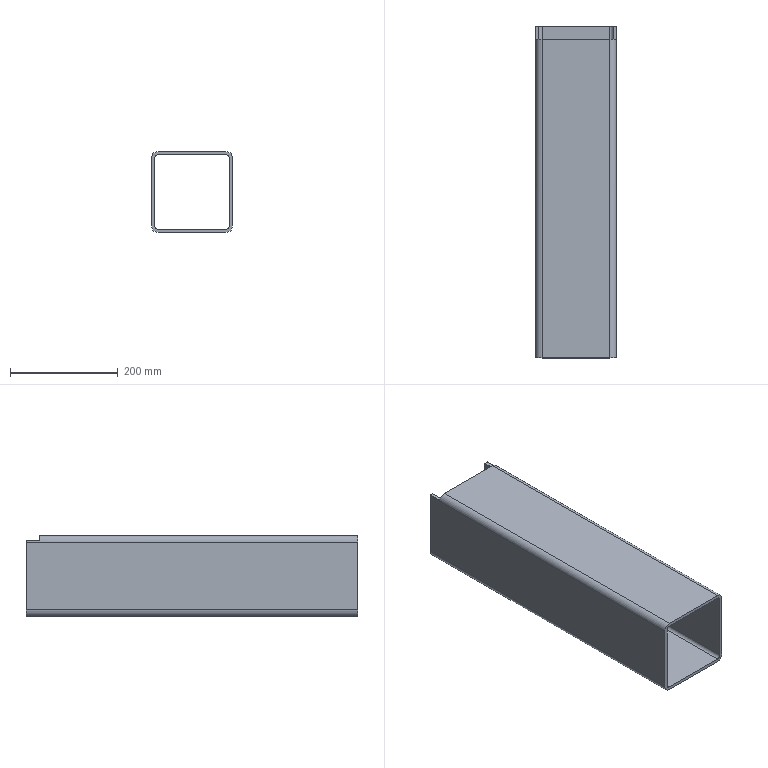Component | SolidWorks | Link2-12 | 1 solid | 21 faces | box 150 x 615 x 150 mm | volume 2045889 mm3 | plane 13 | cylinder 8 | commonest cylinder face diameters 24 x4 12 x4 | material Plain Carbon Steel
build123d program:
from build123d import *

# Parameters (mm, degrees)
BOSS_EXTRUDE1_DEPTH = 615
SKETCH3_W           = 150
SKETCH3_H           = 25
CUT_EXTRUDE1_DEPTH  = 10


with BuildPart() as part:
    # Sketch1 → Boss-Extrude1 (new body)
    with BuildSketch(Plane.XY):
        with BuildLine():
            Line((-63, -75), (63, -75))
            ThreePointArc((63, -75), (71.485, -71.485), (75, -63))
            Line((75, -63), (75, 63))
            ThreePointArc((75, 63), (71.485, 71.485), (63, 75))
            Line((63, 75), (-63, 75))
            ThreePointArc((-63, 75), (-71.485, 71.485), (-75, 63))
            Line((-75, 63), (-75, -63))
            ThreePointArc((-75, -63), (-71.485, -71.485), (-63, -75))
        make_face()
        with BuildLine():
            Line((-63, -69), (63, -69))
            ThreePointArc((63, -69), (67.243, -67.243), (69, -63))
            Line((69, -63), (69, 63))
            ThreePointArc((69, 63), (67.243, 67.243), (63, 69))
            Line((63, 69), (-63, 69))
            ThreePointArc((-63, 69), (-67.243, 67.243), (-69, 63))
            Line((-69, 63), (-69, -63))
            ThreePointArc((-69, -63), (-67.243, -67.243), (-63, -69))
        make_face(mode=Mode.SUBTRACT)
    extrude(amount=BOSS_EXTRUDE1_DEPTH)

    # Sketch3 → Cut-Extrude1 (cut)
    with BuildSketch(Plane(origin=(0, 75, 0), x_dir=(1, 0, 0), z_dir=(0, 1, 0))):
        with Locations((0, -12.5)):
            Rectangle(SKETCH3_W, SKETCH3_H)
    extrude(amount=-CUT_EXTRUDE1_DEPTH, mode=Mode.SUBTRACT)


solid = part.part

# Placed as in the assembly
solid = solid.moved(Location((6192.801, 221.323, 5500.973), (90, 0, 0)))
STEP:
#1=COLOUR_RGB('',0.7922,0.8196,0.9333);
#2=FILL_AREA_STYLE_COLOUR('',#1);
#3=FILL_AREA_STYLE('',(#2));
#4=SURFACE_STYLE_FILL_AREA(#3);
#5=SURFACE_SIDE_STYLE('',(#4));
#6=SURFACE_STYLE_USAGE(.BOTH.,#5);
#7=PRESENTATION_STYLE_ASSIGNMENT((#6));
#8=CARTESIAN_POINT('',(246.757,8.713,219.133));
#9=VERTEX_POINT('',#8);
#10=CARTESIAN_POINT('',(246.514,8.713,219.133));
#11=VERTEX_POINT('',#10);
#12=CARTESIAN_POINT('',(240.858,8.713,219.133));
#13=DIRECTION('',(-1.,0.,0.));
#14=VECTOR('',#13,39.37);
#15=LINE('',#12,#14);
#16=EDGE_CURVE('',#9,#11,#15,.T.);
#17=ORIENTED_EDGE('',*,*,#16,.F.);
#18=CARTESIAN_POINT('',(246.764,8.713,219.054));
#19=VERTEX_POINT('',#18);
#20=CARTESIAN_POINT('',(246.291,8.713,219.054));
#21=DIRECTION('',(0.,-1.,-0.));
#22=DIRECTION('',(1.,0.,0.));
#23=AXIS2_PLACEMENT_3D('',#20,#21,#22);
#24=CIRCLE('',#23,0.4724);
#25=EDGE_CURVE('',#19,#9,#24,.T.);
#26=ORIENTED_EDGE('',*,*,#25,.F.);
#27=CARTESIAN_POINT('',(246.764,8.713,214.093));
#28=VERTEX_POINT('',#27);
#29=CARTESIAN_POINT('',(246.764,8.713,219.054));
#30=DIRECTION('',(0.,0.,-1.));
#31=VECTOR('',#30,39.37);
#32=LINE('',#29,#31);
#33=EDGE_CURVE('',#19,#28,#32,.T.);
#34=ORIENTED_EDGE('',*,*,#33,.T.);
#35=CARTESIAN_POINT('',(246.291,8.713,213.621));
#36=VERTEX_POINT('',#35);
#37=CARTESIAN_POINT('',(246.291,8.713,214.093));
#38=DIRECTION('',(0.,-1.,-0.));
#39=DIRECTION('',(1.,0.,0.));
#40=AXIS2_PLACEMENT_3D('',#37,#38,#39);
#41=CIRCLE('',#40,0.4724);
#42=EDGE_CURVE('',#36,#28,#41,.T.);
#43=ORIENTED_EDGE('',*,*,#42,.F.);
#44=CARTESIAN_POINT('',(241.331,8.713,213.621));
#45=VERTEX_POINT('',#44);
#46=CARTESIAN_POINT('',(241.331,8.713,213.621));
#47=DIRECTION('',(1.,0.,0.));
#48=VECTOR('',#47,39.37);
#49=LINE('',#46,#48);
#50=EDGE_CURVE('',#45,#36,#49,.T.);
#51=ORIENTED_EDGE('',*,*,#50,.F.);
#52=CARTESIAN_POINT('',(240.858,8.713,214.093));
#53=VERTEX_POINT('',#52);
#54=CARTESIAN_POINT('',(241.331,8.713,214.093));
#55=DIRECTION('',(0.,-1.,-0.));
#56=DIRECTION('',(1.,0.,0.));
#57=AXIS2_PLACEMENT_3D('',#54,#55,#56);
#58=CIRCLE('',#57,0.4724);
#59=EDGE_CURVE('',#53,#45,#58,.T.);
#60=ORIENTED_EDGE('',*,*,#59,.F.);
#61=CARTESIAN_POINT('',(240.858,8.713,219.054));
#62=VERTEX_POINT('',#61);
#63=CARTESIAN_POINT('',(240.858,8.713,214.093));
#64=DIRECTION('',(0.,-0.,1.));
#65=VECTOR('',#64,39.37);
#66=LINE('',#63,#65);
#67=EDGE_CURVE('',#53,#62,#66,.T.);
#68=ORIENTED_EDGE('',*,*,#67,.T.);
#69=CARTESIAN_POINT('',(240.865,8.713,219.133));
#70=VERTEX_POINT('',#69);
#71=CARTESIAN_POINT('',(241.331,8.713,219.054));
#72=DIRECTION('',(0.,-1.,-0.));
#73=DIRECTION('',(1.,0.,0.));
#74=AXIS2_PLACEMENT_3D('',#71,#72,#73);
#75=CIRCLE('',#74,0.4724);
#76=EDGE_CURVE('',#70,#62,#75,.T.);
#77=ORIENTED_EDGE('',*,*,#76,.F.);
#78=CARTESIAN_POINT('',(241.108,8.713,219.133));
#79=VERTEX_POINT('',#78);
#80=CARTESIAN_POINT('',(240.858,8.713,219.133));
#81=DIRECTION('',(-1.,0.,0.));
#82=VECTOR('',#81,39.37);
#83=LINE('',#80,#82);
#84=EDGE_CURVE('',#79,#70,#83,.T.);
#85=ORIENTED_EDGE('',*,*,#84,.F.);
#86=CARTESIAN_POINT('',(241.095,8.713,219.054));
#87=VERTEX_POINT('',#86);
#88=CARTESIAN_POINT('',(241.331,8.713,219.054));
#89=DIRECTION('',(0.,-1.,-0.));
#90=DIRECTION('',(1.,0.,0.));
#91=AXIS2_PLACEMENT_3D('',#88,#89,#90);
#92=CIRCLE('',#91,0.2362);
#93=EDGE_CURVE('',#79,#87,#92,.T.);
#94=ORIENTED_EDGE('',*,*,#93,.T.);
#95=CARTESIAN_POINT('',(241.095,8.713,214.093));
#96=VERTEX_POINT('',#95);
#97=CARTESIAN_POINT('',(241.095,8.713,214.093));
#98=DIRECTION('',(0.,-0.,1.));
#99=VECTOR('',#98,39.37);
#100=LINE('',#97,#99);
#101=EDGE_CURVE('',#96,#87,#100,.T.);
#102=ORIENTED_EDGE('',*,*,#101,.F.);
#103=CARTESIAN_POINT('',(241.331,8.713,213.857));
#104=VERTEX_POINT('',#103);
#105=CARTESIAN_POINT('',(241.331,8.713,214.093));
#106=DIRECTION('',(0.,-1.,-0.));
#107=DIRECTION('',(1.,0.,0.));
#108=AXIS2_PLACEMENT_3D('',#105,#106,#107);
#109=CIRCLE('',#108,0.2362);
#110=EDGE_CURVE('',#96,#104,#109,.T.);
#111=ORIENTED_EDGE('',*,*,#110,.T.);
#112=CARTESIAN_POINT('',(246.291,8.713,213.857));
#113=VERTEX_POINT('',#112);
#114=CARTESIAN_POINT('',(241.331,8.713,213.857));
#115=DIRECTION('',(1.,0.,0.));
#116=VECTOR('',#115,39.37);
#117=LINE('',#114,#116);
#118=EDGE_CURVE('',#104,#113,#117,.T.);
#119=ORIENTED_EDGE('',*,*,#118,.T.);
#120=CARTESIAN_POINT('',(246.528,8.713,214.093));
#121=VERTEX_POINT('',#120);
#122=CARTESIAN_POINT('',(246.291,8.713,214.093));
#123=DIRECTION('',(0.,-1.,-0.));
#124=DIRECTION('',(1.,0.,0.));
#125=AXIS2_PLACEMENT_3D('',#122,#123,#124);
#126=CIRCLE('',#125,0.2362);
#127=EDGE_CURVE('',#113,#121,#126,.T.);
#128=ORIENTED_EDGE('',*,*,#127,.T.);
#129=CARTESIAN_POINT('',(246.528,8.713,219.054));
#130=VERTEX_POINT('',#129);
#131=CARTESIAN_POINT('',(246.528,8.713,219.054));
#132=DIRECTION('',(0.,0.,-1.));
#133=VECTOR('',#132,39.37);
#134=LINE('',#131,#133);
#135=EDGE_CURVE('',#130,#121,#134,.T.);
#136=ORIENTED_EDGE('',*,*,#135,.F.);
#137=CARTESIAN_POINT('',(246.291,8.713,219.054));
#138=DIRECTION('',(0.,-1.,-0.));
#139=DIRECTION('',(1.,0.,0.));
#140=AXIS2_PLACEMENT_3D('',#137,#138,#139);
#141=CIRCLE('',#140,0.2362);
#142=EDGE_CURVE('',#130,#11,#141,.T.);
#143=ORIENTED_EDGE('',*,*,#142,.T.);
#144=EDGE_LOOP('',(#17,#26,#34,#43,#51,#60,#68,#77,#85,#94,#102,#111,#119,#128,#136,#143));
#145=FACE_OUTER_BOUND('',#144,.T.);
#146=CARTESIAN_POINT('',(246.291,8.713,219.054));
#147=DIRECTION('',(0.,-1.,-0.));
#148=DIRECTION('',(1.,0.,0.));
#149=AXIS2_PLACEMENT_3D('',#146,#147,#148);
#150=PLANE('',#149);
#151=ADVANCED_FACE('',(#145),#150,.F.);
#152=CARTESIAN_POINT('',(246.764,-15.499,219.054));
#153=VERTEX_POINT('',#152);
#154=CARTESIAN_POINT('',(246.291,-15.499,219.527));
#155=VERTEX_POINT('',#154);
#156=CARTESIAN_POINT('',(246.291,-15.499,219.054));
#157=DIRECTION('',(0.,-1.,-0.));
#158=DIRECTION('',(1.,0.,0.));
#159=AXIS2_PLACEMENT_3D('',#156,#157,#158);
#160=CIRCLE('',#159,0.4724);
#161=EDGE_CURVE('',#153,#155,#160,.T.);
#162=ORIENTED_EDGE('',*,*,#161,.T.);
#163=CARTESIAN_POINT('',(241.331,-15.499,219.527));
#164=VERTEX_POINT('',#163);
#165=CARTESIAN_POINT('',(246.291,-15.499,219.527));
#166=DIRECTION('',(-1.,0.,0.));
#167=VECTOR('',#166,39.37);
#168=LINE('',#165,#167);
#169=EDGE_CURVE('',#155,#164,#168,.T.);
#170=ORIENTED_EDGE('',*,*,#169,.T.);
#171=CARTESIAN_POINT('',(240.858,-15.499,219.054));
#172=VERTEX_POINT('',#171);
#173=CARTESIAN_POINT('',(241.331,-15.499,219.054));
#174=DIRECTION('',(0.,-1.,-0.));
#175=DIRECTION('',(1.,0.,0.));
#176=AXIS2_PLACEMENT_3D('',#173,#174,#175);
#177=CIRCLE('',#176,0.4724);
#178=EDGE_CURVE('',#164,#172,#177,.T.);
#179=ORIENTED_EDGE('',*,*,#178,.T.);
#180=CARTESIAN_POINT('',(240.858,-15.499,214.093));
#181=VERTEX_POINT('',#180);
#182=CARTESIAN_POINT('',(240.858,-15.499,214.093));
#183=DIRECTION('',(0.,-0.,1.));
#184=VECTOR('',#183,39.37);
#185=LINE('',#182,#184);
#186=EDGE_CURVE('',#181,#172,#185,.T.);
#187=ORIENTED_EDGE('',*,*,#186,.F.);
#188=CARTESIAN_POINT('',(241.331,-15.499,213.621));
#189=VERTEX_POINT('',#188);
#190=CARTESIAN_POINT('',(241.331,-15.499,214.093));
#191=DIRECTION('',(0.,-1.,-0.));
#192=DIRECTION('',(1.,0.,0.));
#193=AXIS2_PLACEMENT_3D('',#190,#191,#192);
#194=CIRCLE('',#193,0.4724);
#195=EDGE_CURVE('',#181,#189,#194,.T.);
#196=ORIENTED_EDGE('',*,*,#195,.T.);
#197=CARTESIAN_POINT('',(246.291,-15.499,213.621));
#198=VERTEX_POINT('',#197);
#199=CARTESIAN_POINT('',(241.331,-15.499,213.621));
#200=DIRECTION('',(1.,0.,0.));
#201=VECTOR('',#200,39.37);
#202=LINE('',#199,#201);
#203=EDGE_CURVE('',#189,#198,#202,.T.);
#204=ORIENTED_EDGE('',*,*,#203,.T.);
#205=CARTESIAN_POINT('',(246.764,-15.499,214.093));
#206=VERTEX_POINT('',#205);
#207=CARTESIAN_POINT('',(246.291,-15.499,214.093));
#208=DIRECTION('',(0.,-1.,-0.));
#209=DIRECTION('',(1.,0.,0.));
#210=AXIS2_PLACEMENT_3D('',#207,#208,#209);
#211=CIRCLE('',#210,0.4724);
#212=EDGE_CURVE('',#198,#206,#211,.T.);
#213=ORIENTED_EDGE('',*,*,#212,.T.);
#214=CARTESIAN_POINT('',(246.764,-15.499,219.054));
#215=DIRECTION('',(0.,0.,-1.));
#216=VECTOR('',#215,39.37);
#217=LINE('',#214,#216);
#218=EDGE_CURVE('',#153,#206,#217,.T.);
#219=ORIENTED_EDGE('',*,*,#218,.F.);
#220=EDGE_LOOP('',(#162,#170,#179,#187,#196,#204,#213,#219));
#221=FACE_OUTER_BOUND('',#220,.T.);
#222=CARTESIAN_POINT('',(241.331,-15.499,213.857));
#223=VERTEX_POINT('',#222);
#224=CARTESIAN_POINT('',(246.291,-15.499,213.857));
#225=VERTEX_POINT('',#224);
#226=CARTESIAN_POINT('',(241.331,-15.499,213.857));
#227=DIRECTION('',(1.,0.,0.));
#228=VECTOR('',#227,39.37);
#229=LINE('',#226,#228);
#230=EDGE_CURVE('',#223,#225,#229,.T.);
#231=ORIENTED_EDGE('',*,*,#230,.F.);
#232=CARTESIAN_POINT('',(241.095,-15.499,214.093));
#233=VERTEX_POINT('',#232);
#234=CARTESIAN_POINT('',(241.331,-15.499,214.093));
#235=DIRECTION('',(0.,-1.,-0.));
#236=DIRECTION('',(1.,0.,0.));
#237=AXIS2_PLACEMENT_3D('',#234,#235,#236);
#238=CIRCLE('',#237,0.2362);
#239=EDGE_CURVE('',#233,#223,#238,.T.);
#240=ORIENTED_EDGE('',*,*,#239,.F.);
#241=CARTESIAN_POINT('',(241.095,-15.499,219.054));
#242=VERTEX_POINT('',#241);
#243=CARTESIAN_POINT('',(241.095,-15.499,214.093));
#244=DIRECTION('',(0.,-0.,1.));
#245=VECTOR('',#244,39.37);
#246=LINE('',#243,#245);
#247=EDGE_CURVE('',#233,#242,#246,.T.);
#248=ORIENTED_EDGE('',*,*,#247,.T.);
#249=CARTESIAN_POINT('',(241.331,-15.499,219.29));
#250=VERTEX_POINT('',#249);
#251=CARTESIAN_POINT('',(241.331,-15.499,219.054));
#252=DIRECTION('',(0.,-1.,-0.));
#253=DIRECTION('',(1.,0.,0.));
#254=AXIS2_PLACEMENT_3D('',#251,#252,#253);
#255=CIRCLE('',#254,0.2362);
#256=EDGE_CURVE('',#250,#242,#255,.T.);
#257=ORIENTED_EDGE('',*,*,#256,.F.);
#258=CARTESIAN_POINT('',(246.291,-15.499,219.29));
#259=VERTEX_POINT('',#258);
#260=CARTESIAN_POINT('',(246.291,-15.499,219.29));
#261=DIRECTION('',(-1.,0.,0.));
#262=VECTOR('',#261,39.37);
#263=LINE('',#260,#262);
#264=EDGE_CURVE('',#259,#250,#263,.T.);
#265=ORIENTED_EDGE('',*,*,#264,.F.);
#266=CARTESIAN_POINT('',(246.528,-15.499,219.054));
#267=VERTEX_POINT('',#266);
#268=CARTESIAN_POINT('',(246.291,-15.499,219.054));
#269=DIRECTION('',(0.,-1.,-0.));
#270=DIRECTION('',(1.,0.,0.));
#271=AXIS2_PLACEMENT_3D('',#268,#269,#270);
#272=CIRCLE('',#271,0.2362);
#273=EDGE_CURVE('',#267,#259,#272,.T.);
#274=ORIENTED_EDGE('',*,*,#273,.F.);
#275=CARTESIAN_POINT('',(246.528,-15.499,214.093));
#276=VERTEX_POINT('',#275);
#277=CARTESIAN_POINT('',(246.528,-15.499,219.054));
#278=DIRECTION('',(0.,0.,-1.));
#279=VECTOR('',#278,39.37);
#280=LINE('',#277,#279);
#281=EDGE_CURVE('',#267,#276,#280,.T.);
#282=ORIENTED_EDGE('',*,*,#281,.T.);
#283=CARTESIAN_POINT('',(246.291,-15.499,214.093));
#284=DIRECTION('',(0.,-1.,-0.));
#285=DIRECTION('',(1.,0.,0.));
#286=AXIS2_PLACEMENT_3D('',#283,#284,#285);
#287=CIRCLE('',#286,0.2362);
#288=EDGE_CURVE('',#225,#276,#287,.T.);
#289=ORIENTED_EDGE('',*,*,#288,.F.);
#290=EDGE_LOOP('',(#231,#240,#248,#257,#265,#274,#282,#289));
#291=FACE_BOUND('',#290,.T.);
#292=CARTESIAN_POINT('',(246.291,-15.499,219.054));
#293=DIRECTION('',(0.,-1.,-0.));
#294=DIRECTION('',(1.,0.,0.));
#295=AXIS2_PLACEMENT_3D('',#292,#293,#294);
#296=PLANE('',#295);
#297=ADVANCED_FACE('',(#221,#291),#296,.T.);
#298=CARTESIAN_POINT('',(246.757,7.729,219.133));
#299=VERTEX_POINT('',#298);
#300=CARTESIAN_POINT('',(246.757,-15.499,219.133));
#301=DIRECTION('',(0.,1.,0.));
#302=VECTOR('',#301,39.37);
#303=LINE('',#300,#302);
#304=EDGE_CURVE('',#299,#9,#303,.T.);
#305=ORIENTED_EDGE('',*,*,#304,.F.);
#306=CARTESIAN_POINT('',(246.291,7.729,219.527));
#307=VERTEX_POINT('',#306);
#308=CARTESIAN_POINT('',(246.291,7.729,219.054));
#309=DIRECTION('',(0.,-1.,-0.));
#310=DIRECTION('',(1.,0.,0.));
#311=AXIS2_PLACEMENT_3D('',#308,#309,#310);
#312=CIRCLE('',#311,0.4724);
#313=EDGE_CURVE('',#299,#307,#312,.T.);
#314=ORIENTED_EDGE('',*,*,#313,.T.);
#315=CARTESIAN_POINT('',(246.291,-15.499,219.527));
#316=DIRECTION('',(0.,1.,0.));
#317=VECTOR('',#316,39.37);
#318=LINE('',#315,#317);
#319=EDGE_CURVE('',#155,#307,#318,.T.);
#320=ORIENTED_EDGE('',*,*,#319,.F.);
#321=ORIENTED_EDGE('',*,*,#161,.F.);
#322=CARTESIAN_POINT('',(246.764,-15.499,219.054));
#323=DIRECTION('',(0.,1.,0.));
#324=VECTOR('',#323,39.37);
#325=LINE('',#322,#324);
#326=EDGE_CURVE('',#153,#19,#325,.T.);
#327=ORIENTED_EDGE('',*,*,#326,.T.);
#328=ORIENTED_EDGE('',*,*,#25,.T.);
#329=EDGE_LOOP('',(#305,#314,#320,#321,#327,#328));
#330=FACE_OUTER_BOUND('',#329,.T.);
#331=CARTESIAN_POINT('',(246.291,-15.499,219.054));
#332=DIRECTION('',(0.,1.,0.));
#333=DIRECTION('',(-1.,0.,0.));
#334=AXIS2_PLACEMENT_3D('',#331,#332,#333);
#335=CYLINDRICAL_SURFACE('',#334,0.4724);
#336=ADVANCED_FACE('',(#330),#335,.T.);
#337=ORIENTED_EDGE('',*,*,#319,.T.);
#338=CARTESIAN_POINT('',(241.331,7.729,219.527));
#339=VERTEX_POINT('',#338);
#340=CARTESIAN_POINT('',(240.858,7.729,219.527));
#341=DIRECTION('',(1.,0.,0.));
#342=VECTOR('',#341,39.37);
#343=LINE('',#340,#342);
#344=EDGE_CURVE('',#339,#307,#343,.T.);
#345=ORIENTED_EDGE('',*,*,#344,.F.);
#346=CARTESIAN_POINT('',(241.331,-15.499,219.527));
#347=DIRECTION('',(0.,1.,0.));
#348=VECTOR('',#347,39.37);
#349=LINE('',#346,#348);
#350=EDGE_CURVE('',#164,#339,#349,.T.);
#351=ORIENTED_EDGE('',*,*,#350,.F.);
#352=ORIENTED_EDGE('',*,*,#169,.F.);
#353=EDGE_LOOP('',(#337,#345,#351,#352));
#354=FACE_OUTER_BOUND('',#353,.T.);
#355=CARTESIAN_POINT('',(246.291,-15.499,219.527));
#356=DIRECTION('',(0.,0.,-1.));
#357=DIRECTION('',(0.,1.,0.));
#358=AXIS2_PLACEMENT_3D('',#355,#356,#357);
#359=PLANE('',#358);
#360=ADVANCED_FACE('',(#354),#359,.F.);
#361=ORIENTED_EDGE('',*,*,#350,.T.);
#362=CARTESIAN_POINT('',(240.865,7.729,219.133));
#363=VERTEX_POINT('',#362);
#364=CARTESIAN_POINT('',(241.331,7.729,219.054));
#365=DIRECTION('',(0.,-1.,-0.));
#366=DIRECTION('',(1.,0.,0.));
#367=AXIS2_PLACEMENT_3D('',#364,#365,#366);
#368=CIRCLE('',#367,0.4724);
#369=EDGE_CURVE('',#339,#363,#368,.T.);
#370=ORIENTED_EDGE('',*,*,#369,.T.);
#371=CARTESIAN_POINT('',(240.865,-15.499,219.133));
#372=DIRECTION('',(0.,-1.,-0.));
#373=VECTOR('',#372,39.37);
#374=LINE('',#371,#373);
#375=EDGE_CURVE('',#70,#363,#374,.T.);
#376=ORIENTED_EDGE('',*,*,#375,.F.);
#377=ORIENTED_EDGE('',*,*,#76,.T.);
#378=CARTESIAN_POINT('',(240.858,-15.499,219.054));
#379=DIRECTION('',(0.,1.,0.));
#380=VECTOR('',#379,39.37);
#381=LINE('',#378,#380);
#382=EDGE_CURVE('',#172,#62,#381,.T.);
#383=ORIENTED_EDGE('',*,*,#382,.F.);
#384=ORIENTED_EDGE('',*,*,#178,.F.);
#385=EDGE_LOOP('',(#361,#370,#376,#377,#383,#384));
#386=FACE_OUTER_BOUND('',#385,.T.);
#387=CARTESIAN_POINT('',(241.331,-15.499,219.054));
#388=DIRECTION('',(0.,1.,0.));
#389=DIRECTION('',(-1.,0.,0.));
#390=AXIS2_PLACEMENT_3D('',#387,#388,#389);
#391=CYLINDRICAL_SURFACE('',#390,0.4724);
#392=ADVANCED_FACE('',(#386),#391,.T.);
#393=ORIENTED_EDGE('',*,*,#67,.F.);
#394=CARTESIAN_POINT('',(240.858,-15.499,214.093));
#395=DIRECTION('',(0.,1.,0.));
#396=VECTOR('',#395,39.37);
#397=LINE('',#394,#396);
#398=EDGE_CURVE('',#181,#53,#397,.T.);
#399=ORIENTED_EDGE('',*,*,#398,.F.);
#400=ORIENTED_EDGE('',*,*,#186,.T.);
#401=ORIENTED_EDGE('',*,*,#382,.T.);
#402=EDGE_LOOP('',(#393,#399,#400,#401));
#403=FACE_OUTER_BOUND('',#402,.T.);
#404=CARTESIAN_POINT('',(240.858,-15.499,214.093));
#405=DIRECTION('',(-1.,0.,0.));
#406=DIRECTION('',(0.,-1.,-0.));
#407=AXIS2_PLACEMENT_3D('',#404,#405,#406);
#408=PLANE('',#407);
#409=ADVANCED_FACE('',(#403),#408,.T.);
#410=ORIENTED_EDGE('',*,*,#59,.T.);
#411=CARTESIAN_POINT('',(241.331,-15.499,213.621));
#412=DIRECTION('',(0.,1.,0.));
#413=VECTOR('',#412,39.37);
#414=LINE('',#411,#413);
#415=EDGE_CURVE('',#189,#45,#414,.T.);
#416=ORIENTED_EDGE('',*,*,#415,.F.);
#417=ORIENTED_EDGE('',*,*,#195,.F.);
#418=ORIENTED_EDGE('',*,*,#398,.T.);
#419=EDGE_LOOP('',(#410,#416,#417,#418));
#420=FACE_OUTER_BOUND('',#419,.T.);
#421=CARTESIAN_POINT('',(241.331,-15.499,214.093));
#422=DIRECTION('',(0.,1.,0.));
#423=DIRECTION('',(-1.,0.,0.));
#424=AXIS2_PLACEMENT_3D('',#421,#422,#423);
#425=CYLINDRICAL_SURFACE('',#424,0.4724);
#426=ADVANCED_FACE('',(#420),#425,.T.);
#427=ORIENTED_EDGE('',*,*,#50,.T.);
#428=CARTESIAN_POINT('',(246.291,-15.499,213.621));
#429=DIRECTION('',(0.,1.,0.));
#430=VECTOR('',#429,39.37);
#431=LINE('',#428,#430);
#432=EDGE_CURVE('',#198,#36,#431,.T.);
#433=ORIENTED_EDGE('',*,*,#432,.F.);
#434=ORIENTED_EDGE('',*,*,#203,.F.);
#435=ORIENTED_EDGE('',*,*,#415,.T.);
#436=EDGE_LOOP('',(#427,#433,#434,#435));
#437=FACE_OUTER_BOUND('',#436,.T.);
#438=CARTESIAN_POINT('',(241.331,-15.499,213.621));
#439=DIRECTION('',(0.,-0.,1.));
#440=DIRECTION('',(0.,-1.,-0.));
#441=AXIS2_PLACEMENT_3D('',#438,#439,#440);
#442=PLANE('',#441);
#443=ADVANCED_FACE('',(#437),#442,.F.);
#444=ORIENTED_EDGE('',*,*,#42,.T.);
#445=CARTESIAN_POINT('',(246.764,-15.499,214.093));
#446=DIRECTION('',(0.,1.,0.));
#447=VECTOR('',#446,39.37);
#448=LINE('',#445,#447);
#449=EDGE_CURVE('',#206,#28,#448,.T.);
#450=ORIENTED_EDGE('',*,*,#449,.F.);
#451=ORIENTED_EDGE('',*,*,#212,.F.);
#452=ORIENTED_EDGE('',*,*,#432,.T.);
#453=EDGE_LOOP('',(#444,#450,#451,#452));
#454=FACE_OUTER_BOUND('',#453,.T.);
#455=CARTESIAN_POINT('',(246.291,-15.499,214.093));
#456=DIRECTION('',(0.,1.,0.));
#457=DIRECTION('',(-1.,0.,0.));
#458=AXIS2_PLACEMENT_3D('',#455,#456,#457);
#459=CYLINDRICAL_SURFACE('',#458,0.4724);
#460=ADVANCED_FACE('',(#454),#459,.T.);
#461=ORIENTED_EDGE('',*,*,#33,.F.);
#462=ORIENTED_EDGE('',*,*,#326,.F.);
#463=ORIENTED_EDGE('',*,*,#218,.T.);
#464=ORIENTED_EDGE('',*,*,#449,.T.);
#465=EDGE_LOOP('',(#461,#462,#463,#464));
#466=FACE_OUTER_BOUND('',#465,.T.);
#467=CARTESIAN_POINT('',(246.764,-15.499,219.054));
#468=DIRECTION('',(1.,0.,0.));
#469=DIRECTION('',(0.,1.,0.));
#470=AXIS2_PLACEMENT_3D('',#467,#468,#469);
#471=PLANE('',#470);
#472=ADVANCED_FACE('',(#466),#471,.T.);
#473=ORIENTED_EDGE('',*,*,#110,.F.);
#474=CARTESIAN_POINT('',(241.095,-15.499,214.093));
#475=DIRECTION('',(0.,1.,0.));
#476=VECTOR('',#475,39.37);
#477=LINE('',#474,#476);
#478=EDGE_CURVE('',#233,#96,#477,.T.);
#479=ORIENTED_EDGE('',*,*,#478,.F.);
#480=ORIENTED_EDGE('',*,*,#239,.T.);
#481=CARTESIAN_POINT('',(241.331,-15.499,213.857));
#482=DIRECTION('',(0.,1.,0.));
#483=VECTOR('',#482,39.37);
#484=LINE('',#481,#483);
#485=EDGE_CURVE('',#223,#104,#484,.T.);
#486=ORIENTED_EDGE('',*,*,#485,.T.);
#487=EDGE_LOOP('',(#473,#479,#480,#486));
#488=FACE_OUTER_BOUND('',#487,.T.);
#489=CARTESIAN_POINT('',(241.331,-15.499,214.093));
#490=DIRECTION('',(0.,1.,0.));
#491=DIRECTION('',(-1.,0.,0.));
#492=AXIS2_PLACEMENT_3D('',#489,#490,#491);
#493=CYLINDRICAL_SURFACE('',#492,0.2362);
#494=ADVANCED_FACE('',(#488),#493,.F.);
#495=ORIENTED_EDGE('',*,*,#118,.F.);
#496=ORIENTED_EDGE('',*,*,#485,.F.);
#497=ORIENTED_EDGE('',*,*,#230,.T.);
#498=CARTESIAN_POINT('',(246.291,-15.499,213.857));
#499=DIRECTION('',(0.,1.,0.));
#500=VECTOR('',#499,39.37);
#501=LINE('',#498,#500);
#502=EDGE_CURVE('',#225,#113,#501,.T.);
#503=ORIENTED_EDGE('',*,*,#502,.T.);
#504=EDGE_LOOP('',(#495,#496,#497,#503));
#505=FACE_OUTER_BOUND('',#504,.T.);
#506=CARTESIAN_POINT('',(241.331,-15.499,213.857));
#507=DIRECTION('',(0.,-0.,1.));
#508=DIRECTION('',(0.,-1.,-0.));
#509=AXIS2_PLACEMENT_3D('',#506,#507,#508);
#510=PLANE('',#509);
#511=ADVANCED_FACE('',(#505),#510,.T.);
#512=ORIENTED_EDGE('',*,*,#127,.F.);
#513=ORIENTED_EDGE('',*,*,#502,.F.);
#514=ORIENTED_EDGE('',*,*,#288,.T.);
#515=CARTESIAN_POINT('',(246.528,-15.499,214.093));
#516=DIRECTION('',(0.,1.,0.));
#517=VECTOR('',#516,39.37);
#518=LINE('',#515,#517);
#519=EDGE_CURVE('',#276,#121,#518,.T.);
#520=ORIENTED_EDGE('',*,*,#519,.T.);
#521=EDGE_LOOP('',(#512,#513,#514,#520));
#522=FACE_OUTER_BOUND('',#521,.T.);
#523=CARTESIAN_POINT('',(246.291,-15.499,214.093));
#524=DIRECTION('',(0.,1.,0.));
#525=DIRECTION('',(-1.,0.,0.));
#526=AXIS2_PLACEMENT_3D('',#523,#524,#525);
#527=CYLINDRICAL_SURFACE('',#526,0.2362);
#528=ADVANCED_FACE('',(#522),#527,.F.);
#529=ORIENTED_EDGE('',*,*,#135,.T.);
#530=ORIENTED_EDGE('',*,*,#519,.F.);
#531=ORIENTED_EDGE('',*,*,#281,.F.);
#532=CARTESIAN_POINT('',(246.528,-15.499,219.054));
#533=DIRECTION('',(0.,1.,0.));
#534=VECTOR('',#533,39.37);
#535=LINE('',#532,#534);
#536=EDGE_CURVE('',#267,#130,#535,.T.);
#537=ORIENTED_EDGE('',*,*,#536,.T.);
#538=EDGE_LOOP('',(#529,#530,#531,#537));
#539=FACE_OUTER_BOUND('',#538,.T.);
#540=CARTESIAN_POINT('',(246.528,-15.499,219.054));
#541=DIRECTION('',(1.,0.,0.));
#542=DIRECTION('',(0.,1.,0.));
#543=AXIS2_PLACEMENT_3D('',#540,#541,#542);
#544=PLANE('',#543);
#545=ADVANCED_FACE('',(#539),#544,.F.);
#546=CARTESIAN_POINT('',(246.514,7.729,219.133));
#547=VERTEX_POINT('',#546);
#548=CARTESIAN_POINT('',(246.291,7.729,219.29));
#549=VERTEX_POINT('',#548);
#550=CARTESIAN_POINT('',(246.291,7.729,219.054));
#551=DIRECTION('',(0.,-1.,-0.));
#552=DIRECTION('',(1.,0.,0.));
#553=AXIS2_PLACEMENT_3D('',#550,#551,#552);
#554=CIRCLE('',#553,0.2362);
#555=EDGE_CURVE('',#547,#549,#554,.T.);
#556=ORIENTED_EDGE('',*,*,#555,.F.);
#557=CARTESIAN_POINT('',(246.514,-15.499,219.133));
#558=DIRECTION('',(0.,1.,0.));
#559=VECTOR('',#558,39.37);
#560=LINE('',#557,#559);
#561=EDGE_CURVE('',#547,#11,#560,.T.);
#562=ORIENTED_EDGE('',*,*,#561,.T.);
#563=ORIENTED_EDGE('',*,*,#142,.F.);
#564=ORIENTED_EDGE('',*,*,#536,.F.);
#565=ORIENTED_EDGE('',*,*,#273,.T.);
#566=CARTESIAN_POINT('',(246.291,-15.499,219.29));
#567=DIRECTION('',(0.,1.,0.));
#568=VECTOR('',#567,39.37);
#569=LINE('',#566,#568);
#570=EDGE_CURVE('',#259,#549,#569,.T.);
#571=ORIENTED_EDGE('',*,*,#570,.T.);
#572=EDGE_LOOP('',(#556,#562,#563,#564,#565,#571));
#573=FACE_OUTER_BOUND('',#572,.T.);
#574=CARTESIAN_POINT('',(246.291,-15.499,219.054));
#575=DIRECTION('',(0.,1.,0.));
#576=DIRECTION('',(-1.,0.,0.));
#577=AXIS2_PLACEMENT_3D('',#574,#575,#576);
#578=CYLINDRICAL_SURFACE('',#577,0.2362);
#579=ADVANCED_FACE('',(#573),#578,.F.);
#580=CARTESIAN_POINT('',(241.331,7.729,219.29));
#581=VERTEX_POINT('',#580);
#582=CARTESIAN_POINT('',(246.291,7.729,219.29));
#583=DIRECTION('',(-1.,-0.,-0.));
#584=VECTOR('',#583,39.37);
#585=LINE('',#582,#584);
#586=EDGE_CURVE('',#549,#581,#585,.T.);
#587=ORIENTED_EDGE('',*,*,#586,.F.);
#588=ORIENTED_EDGE('',*,*,#570,.F.);
#589=ORIENTED_EDGE('',*,*,#264,.T.);
#590=CARTESIAN_POINT('',(241.331,-15.499,219.29));
#591=DIRECTION('',(0.,1.,0.));
#592=VECTOR('',#591,39.37);
#593=LINE('',#590,#592);
#594=EDGE_CURVE('',#250,#581,#593,.T.);
#595=ORIENTED_EDGE('',*,*,#594,.T.);
#596=EDGE_LOOP('',(#587,#588,#589,#595));
#597=FACE_OUTER_BOUND('',#596,.T.);
#598=CARTESIAN_POINT('',(246.291,-15.499,219.29));
#599=DIRECTION('',(0.,0.,-1.));
#600=DIRECTION('',(0.,1.,0.));
#601=AXIS2_PLACEMENT_3D('',#598,#599,#600);
#602=PLANE('',#601);
#603=ADVANCED_FACE('',(#597),#602,.T.);
#604=CARTESIAN_POINT('',(241.108,7.729,219.133));
#605=VERTEX_POINT('',#604);
#606=CARTESIAN_POINT('',(241.331,7.729,219.054));
#607=DIRECTION('',(0.,-1.,-0.));
#608=DIRECTION('',(1.,0.,0.));
#609=AXIS2_PLACEMENT_3D('',#606,#607,#608);
#610=CIRCLE('',#609,0.2362);
#611=EDGE_CURVE('',#581,#605,#610,.T.);
#612=ORIENTED_EDGE('',*,*,#611,.F.);
#613=ORIENTED_EDGE('',*,*,#594,.F.);
#614=ORIENTED_EDGE('',*,*,#256,.T.);
#615=CARTESIAN_POINT('',(241.095,-15.499,219.054));
#616=DIRECTION('',(0.,1.,0.));
#617=VECTOR('',#616,39.37);
#618=LINE('',#615,#617);
#619=EDGE_CURVE('',#242,#87,#618,.T.);
#620=ORIENTED_EDGE('',*,*,#619,.T.);
#621=ORIENTED_EDGE('',*,*,#93,.F.);
#622=CARTESIAN_POINT('',(241.108,-15.499,219.133));
#623=DIRECTION('',(0.,-1.,-0.));
#624=VECTOR('',#623,39.37);
#625=LINE('',#622,#624);
#626=EDGE_CURVE('',#79,#605,#625,.T.);
#627=ORIENTED_EDGE('',*,*,#626,.T.);
#628=EDGE_LOOP('',(#612,#613,#614,#620,#621,#627));
#629=FACE_OUTER_BOUND('',#628,.T.);
#630=CARTESIAN_POINT('',(241.331,-15.499,219.054));
#631=DIRECTION('',(0.,1.,0.));
#632=DIRECTION('',(-1.,0.,0.));
#633=AXIS2_PLACEMENT_3D('',#630,#631,#632);
#634=CYLINDRICAL_SURFACE('',#633,0.2362);
#635=ADVANCED_FACE('',(#629),#634,.F.);
#636=ORIENTED_EDGE('',*,*,#101,.T.);
#637=ORIENTED_EDGE('',*,*,#619,.F.);
#638=ORIENTED_EDGE('',*,*,#247,.F.);
#639=ORIENTED_EDGE('',*,*,#478,.T.);
#640=EDGE_LOOP('',(#636,#637,#638,#639));
#641=FACE_OUTER_BOUND('',#640,.T.);
#642=CARTESIAN_POINT('',(241.095,-15.499,214.093));
#643=DIRECTION('',(-1.,0.,0.));
#644=DIRECTION('',(0.,-1.,-0.));
#645=AXIS2_PLACEMENT_3D('',#642,#643,#644);
#646=PLANE('',#645);
#647=ADVANCED_FACE('',(#641),#646,.F.);
#648=CARTESIAN_POINT('',(240.858,7.729,219.133));
#649=DIRECTION('',(1.,0.,0.));
#650=VECTOR('',#649,39.37);
#651=LINE('',#648,#650);
#652=EDGE_CURVE('',#547,#299,#651,.T.);
#653=ORIENTED_EDGE('',*,*,#652,.F.);
#654=ORIENTED_EDGE('',*,*,#555,.T.);
#655=ORIENTED_EDGE('',*,*,#586,.T.);
#656=ORIENTED_EDGE('',*,*,#611,.T.);
#657=CARTESIAN_POINT('',(240.858,7.729,219.133));
#658=DIRECTION('',(1.,0.,0.));
#659=VECTOR('',#658,39.37);
#660=LINE('',#657,#659);
#661=EDGE_CURVE('',#363,#605,#660,.T.);
#662=ORIENTED_EDGE('',*,*,#661,.F.);
#663=ORIENTED_EDGE('',*,*,#369,.F.);
#664=ORIENTED_EDGE('',*,*,#344,.T.);
#665=ORIENTED_EDGE('',*,*,#313,.F.);
#666=EDGE_LOOP('',(#653,#654,#655,#656,#662,#663,#664,#665));
#667=FACE_OUTER_BOUND('',#666,.T.);
#668=CARTESIAN_POINT('',(240.858,7.729,219.133));
#669=DIRECTION('',(0.,-1.,-0.));
#670=DIRECTION('',(1.,0.,0.));
#671=AXIS2_PLACEMENT_3D('',#668,#669,#670);
#672=PLANE('',#671);
#673=ADVANCED_FACE('',(#667),#672,.F.);
#674=ORIENTED_EDGE('',*,*,#304,.T.);
#675=ORIENTED_EDGE('',*,*,#16,.T.);
#676=ORIENTED_EDGE('',*,*,#561,.F.);
#677=ORIENTED_EDGE('',*,*,#652,.T.);
#678=EDGE_LOOP('',(#674,#675,#676,#677));
#679=FACE_OUTER_BOUND('',#678,.T.);
#680=CARTESIAN_POINT('',(243.811,8.713,219.133));
#681=DIRECTION('',(0.,-0.,1.));
#682=DIRECTION('',(0.,-1.,-0.));
#683=AXIS2_PLACEMENT_3D('',#680,#681,#682);
#684=PLANE('',#683);
#685=ADVANCED_FACE('',(#679),#684,.T.);
#686=ORIENTED_EDGE('',*,*,#375,.T.);
#687=ORIENTED_EDGE('',*,*,#661,.T.);
#688=ORIENTED_EDGE('',*,*,#626,.F.);
#689=ORIENTED_EDGE('',*,*,#84,.T.);
#690=EDGE_LOOP('',(#686,#687,#688,#689));
#691=FACE_OUTER_BOUND('',#690,.T.);
#692=CARTESIAN_POINT('',(243.811,8.713,219.133));
#693=DIRECTION('',(0.,-0.,1.));
#694=DIRECTION('',(0.,-1.,-0.));
#695=AXIS2_PLACEMENT_3D('',#692,#693,#694);
#696=PLANE('',#695);
#697=ADVANCED_FACE('',(#691),#696,.T.);
#698=CLOSED_SHELL('',(#151,#297,#336,#360,#392,#409,#426,#443,#460,#472,#494,#511,#528,#545,#579,#603,#635,#647,#673,#685,#697));
#699=MANIFOLD_SOLID_BREP('',#698);
#700=STYLED_ITEM('',(#7),#699);
#701=(LENGTH_UNIT()NAMED_UNIT(*)SI_UNIT($,.METRE.));
#702=LENGTH_MEASURE_WITH_UNIT(LENGTH_MEASURE(0.0254),#701);
#703=DIMENSIONAL_EXPONENTS(1.,0.,0.,0.,0.,0.,0.);
#704=(CONVERSION_BASED_UNIT('',#702)LENGTH_UNIT()NAMED_UNIT(#703));
#705=UNCERTAINTY_MEASURE_WITH_UNIT(LENGTH_MEASURE(0.00001),#704,'','');
#706=(NAMED_UNIT(*)PLANE_ANGLE_UNIT()SI_UNIT($,.RADIAN.));
#707=(NAMED_UNIT(*)SI_UNIT($,.STERADIAN.)SOLID_ANGLE_UNIT());
#708=(GEOMETRIC_REPRESENTATION_CONTEXT(3)GLOBAL_UNCERTAINTY_ASSIGNED_CONTEXT((#705))GLOBAL_UNIT_ASSIGNED_CONTEXT((#704,#706,#707))REPRESENTATION_CONTEXT('',''));
#709=MECHANICAL_DESIGN_GEOMETRIC_PRESENTATION_REPRESENTATION('',(#700),#708);
#710=PRESENTATION_LAYER_ASSIGNMENT('','',(#700));
#711=CARTESIAN_POINT('',(0.,0.,0.));
#712=DIRECTION('',(0.,0.,1.));
#713=DIRECTION('',(1.,0.,0.));
#714=AXIS2_PLACEMENT_3D('',#711,#712,#713);
#715=(LENGTH_UNIT()NAMED_UNIT(*)SI_UNIT($,.METRE.));
#716=LENGTH_MEASURE_WITH_UNIT(LENGTH_MEASURE(0.0254),#715);
#717=DIMENSIONAL_EXPONENTS(1.,0.,0.,0.,0.,0.,0.);
#718=(CONVERSION_BASED_UNIT('',#716)LENGTH_UNIT()NAMED_UNIT(#717));
#719=UNCERTAINTY_MEASURE_WITH_UNIT(LENGTH_MEASURE(0.00001),#718,'','');
#720=(NAMED_UNIT(*)PLANE_ANGLE_UNIT()SI_UNIT($,.RADIAN.));
#721=(NAMED_UNIT(*)SI_UNIT($,.STERADIAN.)SOLID_ANGLE_UNIT());
#722=(GEOMETRIC_REPRESENTATION_CONTEXT(3)GLOBAL_UNCERTAINTY_ASSIGNED_CONTEXT((#719))GLOBAL_UNIT_ASSIGNED_CONTEXT((#718,#720,#721))REPRESENTATION_CONTEXT('',''));
#723=ADVANCED_BREP_SHAPE_REPRESENTATION('',(#699,#714),#722);